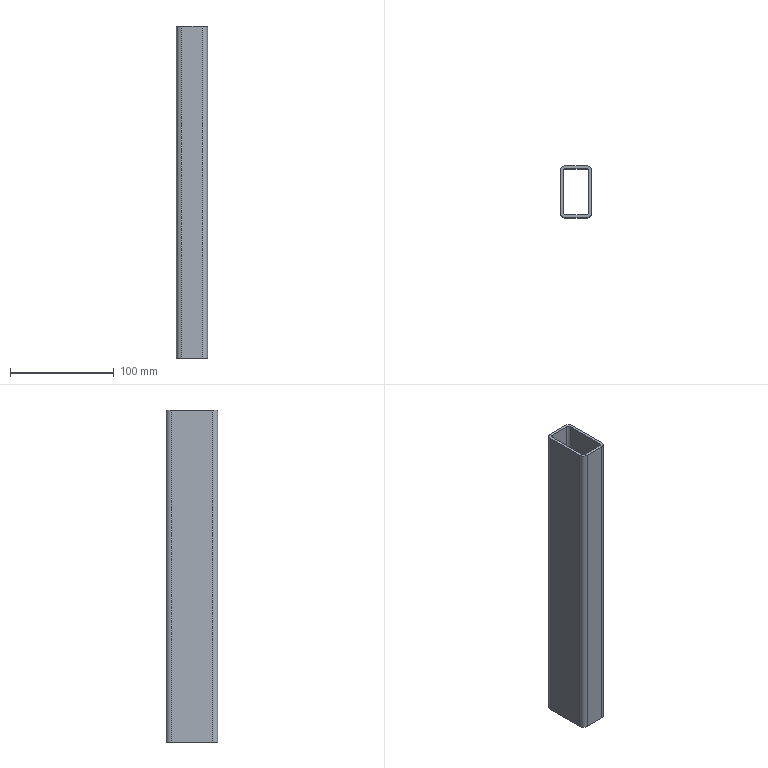Component | SolidWorks | Frame-1_SquareTube13-1 | 1 solid | 18 faces | box 30 x 50 x 320 mm | volume 118896 mm3 | plane 10 | cylinder 8 | commonest cylinder face diameters 5.2 x4 10.4 x4
STEP:
#1=COLOUR_RGB('',0.7922,0.8196,0.9333);
#2=FILL_AREA_STYLE_COLOUR('',#1);
#3=FILL_AREA_STYLE('',(#2));
#4=SURFACE_STYLE_FILL_AREA(#3);
#5=SURFACE_SIDE_STYLE('',(#4));
#6=SURFACE_STYLE_USAGE(.BOTH.,#5);
#7=PRESENTATION_STYLE_ASSIGNMENT((#6));
#8=CARTESIAN_POINT('',(-8.134,-11.622,-6.299));
#9=VERTEX_POINT('',#8);
#10=CARTESIAN_POINT('',(-8.134,-13.181,-6.299));
#11=VERTEX_POINT('',#10);
#12=CARTESIAN_POINT('',(-8.134,-11.622,-6.299));
#13=DIRECTION('',(0.,-1.,0.));
#14=VECTOR('',#13,39.37);
#15=LINE('',#12,#14);
#16=EDGE_CURVE('',#9,#11,#15,.T.);
#17=ORIENTED_EDGE('',*,*,#16,.T.);
#18=CARTESIAN_POINT('',(-8.134,-13.181,6.299));
#19=VERTEX_POINT('',#18);
#20=CARTESIAN_POINT('',(-8.134,-13.181,6.89));
#21=DIRECTION('',(0.,0.,1.));
#22=VECTOR('',#21,39.37);
#23=LINE('',#20,#22);
#24=EDGE_CURVE('',#11,#19,#23,.T.);
#25=ORIENTED_EDGE('',*,*,#24,.T.);
#26=CARTESIAN_POINT('',(-8.134,-11.622,6.299));
#27=VERTEX_POINT('',#26);
#28=CARTESIAN_POINT('',(-8.134,-11.622,6.299));
#29=DIRECTION('',(0.,1.,0.));
#30=VECTOR('',#29,39.37);
#31=LINE('',#28,#30);
#32=EDGE_CURVE('',#19,#27,#31,.T.);
#33=ORIENTED_EDGE('',*,*,#32,.T.);
#34=CARTESIAN_POINT('',(-8.134,-11.622,6.89));
#35=DIRECTION('',(-0.,0.,-1.));
#36=VECTOR('',#35,39.37);
#37=LINE('',#34,#36);
#38=EDGE_CURVE('',#27,#9,#37,.T.);
#39=ORIENTED_EDGE('',*,*,#38,.T.);
#40=EDGE_LOOP('',(#17,#25,#33,#39));
#41=FACE_OUTER_BOUND('',#40,.T.);
#42=CARTESIAN_POINT('',(-8.134,-11.622,6.89));
#43=DIRECTION('',(-1.,0.,0.));
#44=DIRECTION('',(0.,0.,1.));
#45=AXIS2_PLACEMENT_3D('',#42,#43,#44);
#46=PLANE('',#45);
#47=ADVANCED_FACE('',(#41),#46,.T.);
#48=ORIENTED_EDGE('',*,*,#24,.F.);
#49=CARTESIAN_POINT('',(-8.236,-13.283,-6.299));
#50=VERTEX_POINT('',#49);
#51=CARTESIAN_POINT('',(-8.236,-13.181,-6.299));
#52=DIRECTION('',(0.,0.,1.));
#53=DIRECTION('',(-1.,0.,0.));
#54=AXIS2_PLACEMENT_3D('',#51,#52,#53);
#55=CIRCLE('',#54,0.1024);
#56=EDGE_CURVE('',#50,#11,#55,.T.);
#57=ORIENTED_EDGE('',*,*,#56,.F.);
#58=CARTESIAN_POINT('',(-8.236,-13.283,6.299));
#59=VERTEX_POINT('',#58);
#60=CARTESIAN_POINT('',(-8.236,-13.283,6.89));
#61=DIRECTION('',(-0.,0.,-1.));
#62=VECTOR('',#61,39.37);
#63=LINE('',#60,#62);
#64=EDGE_CURVE('',#59,#50,#63,.T.);
#65=ORIENTED_EDGE('',*,*,#64,.F.);
#66=CARTESIAN_POINT('',(-8.236,-13.181,6.299));
#67=DIRECTION('',(-0.,0.,-1.));
#68=DIRECTION('',(-1.,0.,0.));
#69=AXIS2_PLACEMENT_3D('',#66,#67,#68);
#70=CIRCLE('',#69,0.1024);
#71=EDGE_CURVE('',#19,#59,#70,.T.);
#72=ORIENTED_EDGE('',*,*,#71,.F.);
#73=EDGE_LOOP('',(#48,#57,#65,#72));
#74=FACE_OUTER_BOUND('',#73,.T.);
#75=CARTESIAN_POINT('',(-8.236,-13.181,6.89));
#76=DIRECTION('',(-0.,0.,-1.));
#77=DIRECTION('',(-1.,0.,0.));
#78=AXIS2_PLACEMENT_3D('',#75,#76,#77);
#79=CYLINDRICAL_SURFACE('',#78,0.1024);
#80=ADVANCED_FACE('',(#74),#79,.F.);
#81=CARTESIAN_POINT('',(-8.236,-13.386,-6.299));
#82=VERTEX_POINT('',#81);
#83=CARTESIAN_POINT('',(-8.031,-13.181,-6.299));
#84=VERTEX_POINT('',#83);
#85=CARTESIAN_POINT('',(-8.236,-13.181,-6.299));
#86=DIRECTION('',(0.,0.,1.));
#87=DIRECTION('',(-1.,0.,0.));
#88=AXIS2_PLACEMENT_3D('',#85,#86,#87);
#89=CIRCLE('',#88,0.2047);
#90=EDGE_CURVE('',#82,#84,#89,.T.);
#91=ORIENTED_EDGE('',*,*,#90,.F.);
#92=CARTESIAN_POINT('',(-9.008,-13.386,-6.299));
#93=VERTEX_POINT('',#92);
#94=CARTESIAN_POINT('',(0.,-13.386,-6.299));
#95=DIRECTION('',(1.,0.,0.));
#96=VECTOR('',#95,39.37);
#97=LINE('',#94,#96);
#98=EDGE_CURVE('',#93,#82,#97,.T.);
#99=ORIENTED_EDGE('',*,*,#98,.F.);
#100=CARTESIAN_POINT('',(-9.213,-13.181,-6.299));
#101=VERTEX_POINT('',#100);
#102=CARTESIAN_POINT('',(-9.008,-13.181,-6.299));
#103=DIRECTION('',(0.,0.,1.));
#104=DIRECTION('',(-1.,0.,0.));
#105=AXIS2_PLACEMENT_3D('',#102,#103,#104);
#106=CIRCLE('',#105,0.2047);
#107=EDGE_CURVE('',#101,#93,#106,.T.);
#108=ORIENTED_EDGE('',*,*,#107,.F.);
#109=CARTESIAN_POINT('',(-9.213,-11.622,-6.299));
#110=VERTEX_POINT('',#109);
#111=CARTESIAN_POINT('',(-9.213,-12.402,-6.299));
#112=DIRECTION('',(0.,-1.,0.));
#113=VECTOR('',#112,39.37);
#114=LINE('',#111,#113);
#115=EDGE_CURVE('',#110,#101,#114,.T.);
#116=ORIENTED_EDGE('',*,*,#115,.F.);
#117=CARTESIAN_POINT('',(-9.008,-11.417,-6.299));
#118=VERTEX_POINT('',#117);
#119=CARTESIAN_POINT('',(-9.008,-11.622,-6.299));
#120=DIRECTION('',(0.,0.,1.));
#121=DIRECTION('',(-1.,0.,0.));
#122=AXIS2_PLACEMENT_3D('',#119,#120,#121);
#123=CIRCLE('',#122,0.2047);
#124=EDGE_CURVE('',#118,#110,#123,.T.);
#125=ORIENTED_EDGE('',*,*,#124,.F.);
#126=CARTESIAN_POINT('',(-8.236,-11.417,-6.299));
#127=VERTEX_POINT('',#126);
#128=CARTESIAN_POINT('',(0.,-11.417,-6.299));
#129=DIRECTION('',(-1.,0.,0.));
#130=VECTOR('',#129,39.37);
#131=LINE('',#128,#130);
#132=EDGE_CURVE('',#127,#118,#131,.T.);
#133=ORIENTED_EDGE('',*,*,#132,.F.);
#134=CARTESIAN_POINT('',(-8.031,-11.622,-6.299));
#135=VERTEX_POINT('',#134);
#136=CARTESIAN_POINT('',(-8.236,-11.622,-6.299));
#137=DIRECTION('',(0.,0.,1.));
#138=DIRECTION('',(-1.,0.,0.));
#139=AXIS2_PLACEMENT_3D('',#136,#137,#138);
#140=CIRCLE('',#139,0.2047);
#141=EDGE_CURVE('',#135,#127,#140,.T.);
#142=ORIENTED_EDGE('',*,*,#141,.F.);
#143=CARTESIAN_POINT('',(-8.031,-12.402,-6.299));
#144=DIRECTION('',(0.,1.,0.));
#145=VECTOR('',#144,39.37);
#146=LINE('',#143,#145);
#147=EDGE_CURVE('',#84,#135,#146,.T.);
#148=ORIENTED_EDGE('',*,*,#147,.F.);
#149=EDGE_LOOP('',(#91,#99,#108,#116,#125,#133,#142,#148));
#150=FACE_OUTER_BOUND('',#149,.T.);
#151=CARTESIAN_POINT('',(-9.11,-13.181,-6.299));
#152=VERTEX_POINT('',#151);
#153=CARTESIAN_POINT('',(-9.11,-11.622,-6.299));
#154=VERTEX_POINT('',#153);
#155=CARTESIAN_POINT('',(-9.11,-12.402,-6.299));
#156=DIRECTION('',(0.,1.,0.));
#157=VECTOR('',#156,39.37);
#158=LINE('',#155,#157);
#159=EDGE_CURVE('',#152,#154,#158,.T.);
#160=ORIENTED_EDGE('',*,*,#159,.F.);
#161=CARTESIAN_POINT('',(-9.008,-13.283,-6.299));
#162=VERTEX_POINT('',#161);
#163=CARTESIAN_POINT('',(-9.008,-13.181,-6.299));
#164=DIRECTION('',(-0.,0.,-1.));
#165=DIRECTION('',(-1.,0.,0.));
#166=AXIS2_PLACEMENT_3D('',#163,#164,#165);
#167=CIRCLE('',#166,0.1024);
#168=EDGE_CURVE('',#162,#152,#167,.T.);
#169=ORIENTED_EDGE('',*,*,#168,.F.);
#170=CARTESIAN_POINT('',(0.,-13.283,-6.299));
#171=DIRECTION('',(-1.,0.,0.));
#172=VECTOR('',#171,39.37);
#173=LINE('',#170,#172);
#174=EDGE_CURVE('',#50,#162,#173,.T.);
#175=ORIENTED_EDGE('',*,*,#174,.F.);
#176=ORIENTED_EDGE('',*,*,#56,.T.);
#177=ORIENTED_EDGE('',*,*,#16,.F.);
#178=CARTESIAN_POINT('',(-8.236,-11.52,-6.299));
#179=VERTEX_POINT('',#178);
#180=CARTESIAN_POINT('',(-8.236,-11.622,-6.299));
#181=DIRECTION('',(-0.,0.,-1.));
#182=DIRECTION('',(-1.,0.,0.));
#183=AXIS2_PLACEMENT_3D('',#180,#181,#182);
#184=CIRCLE('',#183,0.1024);
#185=EDGE_CURVE('',#179,#9,#184,.T.);
#186=ORIENTED_EDGE('',*,*,#185,.F.);
#187=CARTESIAN_POINT('',(-9.008,-11.52,-6.299));
#188=VERTEX_POINT('',#187);
#189=CARTESIAN_POINT('',(0.,-11.52,-6.299));
#190=DIRECTION('',(1.,0.,0.));
#191=VECTOR('',#190,39.37);
#192=LINE('',#189,#191);
#193=EDGE_CURVE('',#188,#179,#192,.T.);
#194=ORIENTED_EDGE('',*,*,#193,.F.);
#195=CARTESIAN_POINT('',(-9.008,-11.622,-6.299));
#196=DIRECTION('',(-0.,0.,-1.));
#197=DIRECTION('',(-1.,0.,0.));
#198=AXIS2_PLACEMENT_3D('',#195,#196,#197);
#199=CIRCLE('',#198,0.1024);
#200=EDGE_CURVE('',#154,#188,#199,.T.);
#201=ORIENTED_EDGE('',*,*,#200,.F.);
#202=EDGE_LOOP('',(#160,#169,#175,#176,#177,#186,#194,#201));
#203=FACE_BOUND('',#202,.T.);
#204=CARTESIAN_POINT('',(0.,-12.402,-6.299));
#205=DIRECTION('',(0.,0.,1.));
#206=DIRECTION('',(1.,0.,0.));
#207=AXIS2_PLACEMENT_3D('',#204,#205,#206);
#208=PLANE('',#207);
#209=ADVANCED_FACE('',(#150,#203),#208,.F.);
#210=CARTESIAN_POINT('',(-8.236,-11.52,6.299));
#211=VERTEX_POINT('',#210);
#212=CARTESIAN_POINT('',(-8.236,-11.52,6.89));
#213=DIRECTION('',(0.,0.,1.));
#214=VECTOR('',#213,39.37);
#215=LINE('',#212,#214);
#216=EDGE_CURVE('',#179,#211,#215,.T.);
#217=ORIENTED_EDGE('',*,*,#216,.F.);
#218=ORIENTED_EDGE('',*,*,#185,.T.);
#219=ORIENTED_EDGE('',*,*,#38,.F.);
#220=CARTESIAN_POINT('',(-8.236,-11.622,6.299));
#221=DIRECTION('',(-0.,0.,-1.));
#222=DIRECTION('',(-1.,0.,0.));
#223=AXIS2_PLACEMENT_3D('',#220,#221,#222);
#224=CIRCLE('',#223,0.1024);
#225=EDGE_CURVE('',#211,#27,#224,.T.);
#226=ORIENTED_EDGE('',*,*,#225,.F.);
#227=EDGE_LOOP('',(#217,#218,#219,#226));
#228=FACE_OUTER_BOUND('',#227,.T.);
#229=CARTESIAN_POINT('',(-8.236,-11.622,6.89));
#230=DIRECTION('',(-0.,0.,-1.));
#231=DIRECTION('',(-1.,0.,0.));
#232=AXIS2_PLACEMENT_3D('',#229,#230,#231);
#233=CYLINDRICAL_SURFACE('',#232,0.1024);
#234=ADVANCED_FACE('',(#228),#233,.F.);
#235=CARTESIAN_POINT('',(-9.008,-11.417,6.299));
#236=VERTEX_POINT('',#235);
#237=CARTESIAN_POINT('',(-8.236,-11.417,6.299));
#238=VERTEX_POINT('',#237);
#239=CARTESIAN_POINT('',(0.,-11.417,6.299));
#240=DIRECTION('',(1.,0.,0.));
#241=VECTOR('',#240,39.37);
#242=LINE('',#239,#241);
#243=EDGE_CURVE('',#236,#238,#242,.T.);
#244=ORIENTED_EDGE('',*,*,#243,.F.);
#245=CARTESIAN_POINT('',(-9.213,-11.622,6.299));
#246=VERTEX_POINT('',#245);
#247=CARTESIAN_POINT('',(-9.008,-11.622,6.299));
#248=DIRECTION('',(-0.,0.,-1.));
#249=DIRECTION('',(-1.,0.,0.));
#250=AXIS2_PLACEMENT_3D('',#247,#248,#249);
#251=CIRCLE('',#250,0.2047);
#252=EDGE_CURVE('',#246,#236,#251,.T.);
#253=ORIENTED_EDGE('',*,*,#252,.F.);
#254=CARTESIAN_POINT('',(-9.213,-13.181,6.299));
#255=VERTEX_POINT('',#254);
#256=CARTESIAN_POINT('',(-9.213,-12.402,6.299));
#257=DIRECTION('',(0.,1.,0.));
#258=VECTOR('',#257,39.37);
#259=LINE('',#256,#258);
#260=EDGE_CURVE('',#255,#246,#259,.T.);
#261=ORIENTED_EDGE('',*,*,#260,.F.);
#262=CARTESIAN_POINT('',(-9.008,-13.386,6.299));
#263=VERTEX_POINT('',#262);
#264=CARTESIAN_POINT('',(-9.008,-13.181,6.299));
#265=DIRECTION('',(-0.,0.,-1.));
#266=DIRECTION('',(-1.,0.,0.));
#267=AXIS2_PLACEMENT_3D('',#264,#265,#266);
#268=CIRCLE('',#267,0.2047);
#269=EDGE_CURVE('',#263,#255,#268,.T.);
#270=ORIENTED_EDGE('',*,*,#269,.F.);
#271=CARTESIAN_POINT('',(-8.236,-13.386,6.299));
#272=VERTEX_POINT('',#271);
#273=CARTESIAN_POINT('',(0.,-13.386,6.299));
#274=DIRECTION('',(-1.,0.,0.));
#275=VECTOR('',#274,39.37);
#276=LINE('',#273,#275);
#277=EDGE_CURVE('',#272,#263,#276,.T.);
#278=ORIENTED_EDGE('',*,*,#277,.F.);
#279=CARTESIAN_POINT('',(-8.031,-13.181,6.299));
#280=VERTEX_POINT('',#279);
#281=CARTESIAN_POINT('',(-8.236,-13.181,6.299));
#282=DIRECTION('',(-0.,0.,-1.));
#283=DIRECTION('',(-1.,0.,0.));
#284=AXIS2_PLACEMENT_3D('',#281,#282,#283);
#285=CIRCLE('',#284,0.2047);
#286=EDGE_CURVE('',#280,#272,#285,.T.);
#287=ORIENTED_EDGE('',*,*,#286,.F.);
#288=CARTESIAN_POINT('',(-8.031,-11.622,6.299));
#289=VERTEX_POINT('',#288);
#290=CARTESIAN_POINT('',(-8.031,-12.402,6.299));
#291=DIRECTION('',(0.,-1.,0.));
#292=VECTOR('',#291,39.37);
#293=LINE('',#290,#292);
#294=EDGE_CURVE('',#289,#280,#293,.T.);
#295=ORIENTED_EDGE('',*,*,#294,.F.);
#296=CARTESIAN_POINT('',(-8.236,-11.622,6.299));
#297=DIRECTION('',(-0.,0.,-1.));
#298=DIRECTION('',(-1.,0.,0.));
#299=AXIS2_PLACEMENT_3D('',#296,#297,#298);
#300=CIRCLE('',#299,0.2047);
#301=EDGE_CURVE('',#238,#289,#300,.T.);
#302=ORIENTED_EDGE('',*,*,#301,.F.);
#303=EDGE_LOOP('',(#244,#253,#261,#270,#278,#287,#295,#302));
#304=FACE_OUTER_BOUND('',#303,.T.);
#305=CARTESIAN_POINT('',(-9.008,-11.52,6.299));
#306=VERTEX_POINT('',#305);
#307=CARTESIAN_POINT('',(-9.11,-11.622,6.299));
#308=VERTEX_POINT('',#307);
#309=CARTESIAN_POINT('',(-9.008,-11.622,6.299));
#310=DIRECTION('',(0.,0.,1.));
#311=DIRECTION('',(-1.,0.,0.));
#312=AXIS2_PLACEMENT_3D('',#309,#310,#311);
#313=CIRCLE('',#312,0.1024);
#314=EDGE_CURVE('',#306,#308,#313,.T.);
#315=ORIENTED_EDGE('',*,*,#314,.F.);
#316=CARTESIAN_POINT('',(0.,-11.52,6.299));
#317=DIRECTION('',(-1.,0.,0.));
#318=VECTOR('',#317,39.37);
#319=LINE('',#316,#318);
#320=EDGE_CURVE('',#211,#306,#319,.T.);
#321=ORIENTED_EDGE('',*,*,#320,.F.);
#322=ORIENTED_EDGE('',*,*,#225,.T.);
#323=ORIENTED_EDGE('',*,*,#32,.F.);
#324=ORIENTED_EDGE('',*,*,#71,.T.);
#325=CARTESIAN_POINT('',(-9.008,-13.283,6.299));
#326=VERTEX_POINT('',#325);
#327=CARTESIAN_POINT('',(0.,-13.283,6.299));
#328=DIRECTION('',(1.,0.,0.));
#329=VECTOR('',#328,39.37);
#330=LINE('',#327,#329);
#331=EDGE_CURVE('',#326,#59,#330,.T.);
#332=ORIENTED_EDGE('',*,*,#331,.F.);
#333=CARTESIAN_POINT('',(-9.11,-13.181,6.299));
#334=VERTEX_POINT('',#333);
#335=CARTESIAN_POINT('',(-9.008,-13.181,6.299));
#336=DIRECTION('',(0.,0.,1.));
#337=DIRECTION('',(-1.,0.,0.));
#338=AXIS2_PLACEMENT_3D('',#335,#336,#337);
#339=CIRCLE('',#338,0.1024);
#340=EDGE_CURVE('',#334,#326,#339,.T.);
#341=ORIENTED_EDGE('',*,*,#340,.F.);
#342=CARTESIAN_POINT('',(-9.11,-12.402,6.299));
#343=DIRECTION('',(0.,-1.,0.));
#344=VECTOR('',#343,39.37);
#345=LINE('',#342,#344);
#346=EDGE_CURVE('',#308,#334,#345,.T.);
#347=ORIENTED_EDGE('',*,*,#346,.F.);
#348=EDGE_LOOP('',(#315,#321,#322,#323,#324,#332,#341,#347));
#349=FACE_BOUND('',#348,.T.);
#350=CARTESIAN_POINT('',(0.,-12.402,6.299));
#351=DIRECTION('',(0.,0.,-1.));
#352=DIRECTION('',(-1.,0.,0.));
#353=AXIS2_PLACEMENT_3D('',#350,#351,#352);
#354=PLANE('',#353);
#355=ADVANCED_FACE('',(#304,#349),#354,.F.);
#356=ORIENTED_EDGE('',*,*,#174,.T.);
#357=CARTESIAN_POINT('',(-9.008,-13.283,6.89));
#358=DIRECTION('',(0.,0.,1.));
#359=VECTOR('',#358,39.37);
#360=LINE('',#357,#359);
#361=EDGE_CURVE('',#162,#326,#360,.T.);
#362=ORIENTED_EDGE('',*,*,#361,.T.);
#363=ORIENTED_EDGE('',*,*,#331,.T.);
#364=ORIENTED_EDGE('',*,*,#64,.T.);
#365=EDGE_LOOP('',(#356,#362,#363,#364));
#366=FACE_OUTER_BOUND('',#365,.T.);
#367=CARTESIAN_POINT('',(-9.008,-13.283,6.89));
#368=DIRECTION('',(0.,1.,0.));
#369=DIRECTION('',(0.,0.,1.));
#370=AXIS2_PLACEMENT_3D('',#367,#368,#369);
#371=PLANE('',#370);
#372=ADVANCED_FACE('',(#366),#371,.T.);
#373=ORIENTED_EDGE('',*,*,#294,.T.);
#374=CARTESIAN_POINT('',(-8.031,-13.181,6.89));
#375=DIRECTION('',(0.,0.,1.));
#376=VECTOR('',#375,39.37);
#377=LINE('',#374,#376);
#378=EDGE_CURVE('',#84,#280,#377,.T.);
#379=ORIENTED_EDGE('',*,*,#378,.F.);
#380=ORIENTED_EDGE('',*,*,#147,.T.);
#381=CARTESIAN_POINT('',(-8.031,-11.622,6.89));
#382=DIRECTION('',(-0.,0.,-1.));
#383=VECTOR('',#382,39.37);
#384=LINE('',#381,#383);
#385=EDGE_CURVE('',#289,#135,#384,.T.);
#386=ORIENTED_EDGE('',*,*,#385,.F.);
#387=EDGE_LOOP('',(#373,#379,#380,#386));
#388=FACE_OUTER_BOUND('',#387,.T.);
#389=CARTESIAN_POINT('',(-8.031,-11.622,6.89));
#390=DIRECTION('',(-1.,0.,0.));
#391=DIRECTION('',(0.,0.,1.));
#392=AXIS2_PLACEMENT_3D('',#389,#390,#391);
#393=PLANE('',#392);
#394=ADVANCED_FACE('',(#388),#393,.F.);
#395=CARTESIAN_POINT('',(-8.236,-13.386,6.89));
#396=DIRECTION('',(-0.,0.,-1.));
#397=VECTOR('',#396,39.37);
#398=LINE('',#395,#397);
#399=EDGE_CURVE('',#272,#82,#398,.T.);
#400=ORIENTED_EDGE('',*,*,#399,.T.);
#401=ORIENTED_EDGE('',*,*,#90,.T.);
#402=ORIENTED_EDGE('',*,*,#378,.T.);
#403=ORIENTED_EDGE('',*,*,#286,.T.);
#404=EDGE_LOOP('',(#400,#401,#402,#403));
#405=FACE_OUTER_BOUND('',#404,.T.);
#406=CARTESIAN_POINT('',(-8.236,-13.181,6.89));
#407=DIRECTION('',(-0.,0.,-1.));
#408=DIRECTION('',(-1.,0.,0.));
#409=AXIS2_PLACEMENT_3D('',#406,#407,#408);
#410=CYLINDRICAL_SURFACE('',#409,0.2047);
#411=ADVANCED_FACE('',(#405),#410,.T.);
#412=ORIENTED_EDGE('',*,*,#277,.T.);
#413=CARTESIAN_POINT('',(-9.008,-13.386,6.89));
#414=DIRECTION('',(0.,0.,1.));
#415=VECTOR('',#414,39.37);
#416=LINE('',#413,#415);
#417=EDGE_CURVE('',#93,#263,#416,.T.);
#418=ORIENTED_EDGE('',*,*,#417,.F.);
#419=ORIENTED_EDGE('',*,*,#98,.T.);
#420=ORIENTED_EDGE('',*,*,#399,.F.);
#421=EDGE_LOOP('',(#412,#418,#419,#420));
#422=FACE_OUTER_BOUND('',#421,.T.);
#423=CARTESIAN_POINT('',(-9.008,-13.386,6.89));
#424=DIRECTION('',(0.,1.,0.));
#425=DIRECTION('',(0.,0.,1.));
#426=AXIS2_PLACEMENT_3D('',#423,#424,#425);
#427=PLANE('',#426);
#428=ADVANCED_FACE('',(#422),#427,.F.);
#429=CARTESIAN_POINT('',(-9.213,-13.181,6.89));
#430=DIRECTION('',(-0.,0.,-1.));
#431=VECTOR('',#430,39.37);
#432=LINE('',#429,#431);
#433=EDGE_CURVE('',#255,#101,#432,.T.);
#434=ORIENTED_EDGE('',*,*,#433,.T.);
#435=ORIENTED_EDGE('',*,*,#107,.T.);
#436=ORIENTED_EDGE('',*,*,#417,.T.);
#437=ORIENTED_EDGE('',*,*,#269,.T.);
#438=EDGE_LOOP('',(#434,#435,#436,#437));
#439=FACE_OUTER_BOUND('',#438,.T.);
#440=CARTESIAN_POINT('',(-9.008,-13.181,6.89));
#441=DIRECTION('',(-0.,0.,-1.));
#442=DIRECTION('',(-1.,0.,0.));
#443=AXIS2_PLACEMENT_3D('',#440,#441,#442);
#444=CYLINDRICAL_SURFACE('',#443,0.2047);
#445=ADVANCED_FACE('',(#439),#444,.T.);
#446=ORIENTED_EDGE('',*,*,#260,.T.);
#447=CARTESIAN_POINT('',(-9.213,-11.622,6.89));
#448=DIRECTION('',(0.,0.,1.));
#449=VECTOR('',#448,39.37);
#450=LINE('',#447,#449);
#451=EDGE_CURVE('',#110,#246,#450,.T.);
#452=ORIENTED_EDGE('',*,*,#451,.F.);
#453=ORIENTED_EDGE('',*,*,#115,.T.);
#454=ORIENTED_EDGE('',*,*,#433,.F.);
#455=EDGE_LOOP('',(#446,#452,#453,#454));
#456=FACE_OUTER_BOUND('',#455,.T.);
#457=CARTESIAN_POINT('',(-9.213,-13.181,6.89));
#458=DIRECTION('',(1.,0.,-0.));
#459=DIRECTION('',(-0.,0.,-1.));
#460=AXIS2_PLACEMENT_3D('',#457,#458,#459);
#461=PLANE('',#460);
#462=ADVANCED_FACE('',(#456),#461,.F.);
#463=CARTESIAN_POINT('',(-9.008,-11.417,6.89));
#464=DIRECTION('',(-0.,0.,-1.));
#465=VECTOR('',#464,39.37);
#466=LINE('',#463,#465);
#467=EDGE_CURVE('',#236,#118,#466,.T.);
#468=ORIENTED_EDGE('',*,*,#467,.T.);
#469=ORIENTED_EDGE('',*,*,#124,.T.);
#470=ORIENTED_EDGE('',*,*,#451,.T.);
#471=ORIENTED_EDGE('',*,*,#252,.T.);
#472=EDGE_LOOP('',(#468,#469,#470,#471));
#473=FACE_OUTER_BOUND('',#472,.T.);
#474=CARTESIAN_POINT('',(-9.008,-11.622,6.89));
#475=DIRECTION('',(-0.,0.,-1.));
#476=DIRECTION('',(-1.,0.,0.));
#477=AXIS2_PLACEMENT_3D('',#474,#475,#476);
#478=CYLINDRICAL_SURFACE('',#477,0.2047);
#479=ADVANCED_FACE('',(#473),#478,.T.);
#480=ORIENTED_EDGE('',*,*,#243,.T.);
#481=CARTESIAN_POINT('',(-8.236,-11.417,6.89));
#482=DIRECTION('',(0.,0.,1.));
#483=VECTOR('',#482,39.37);
#484=LINE('',#481,#483);
#485=EDGE_CURVE('',#127,#238,#484,.T.);
#486=ORIENTED_EDGE('',*,*,#485,.F.);
#487=ORIENTED_EDGE('',*,*,#132,.T.);
#488=ORIENTED_EDGE('',*,*,#467,.F.);
#489=EDGE_LOOP('',(#480,#486,#487,#488));
#490=FACE_OUTER_BOUND('',#489,.T.);
#491=CARTESIAN_POINT('',(-8.236,-11.417,6.89));
#492=DIRECTION('',(0.,-1.,0.));
#493=DIRECTION('',(0.,0.,-1.));
#494=AXIS2_PLACEMENT_3D('',#491,#492,#493);
#495=PLANE('',#494);
#496=ADVANCED_FACE('',(#490),#495,.F.);
#497=ORIENTED_EDGE('',*,*,#385,.T.);
#498=ORIENTED_EDGE('',*,*,#141,.T.);
#499=ORIENTED_EDGE('',*,*,#485,.T.);
#500=ORIENTED_EDGE('',*,*,#301,.T.);
#501=EDGE_LOOP('',(#497,#498,#499,#500));
#502=FACE_OUTER_BOUND('',#501,.T.);
#503=CARTESIAN_POINT('',(-8.236,-11.622,6.89));
#504=DIRECTION('',(-0.,0.,-1.));
#505=DIRECTION('',(-1.,0.,0.));
#506=AXIS2_PLACEMENT_3D('',#503,#504,#505);
#507=CYLINDRICAL_SURFACE('',#506,0.2047);
#508=ADVANCED_FACE('',(#502),#507,.T.);
#509=CARTESIAN_POINT('',(-9.11,-11.622,6.89));
#510=DIRECTION('',(0.,0.,1.));
#511=VECTOR('',#510,39.37);
#512=LINE('',#509,#511);
#513=EDGE_CURVE('',#154,#308,#512,.T.);
#514=ORIENTED_EDGE('',*,*,#513,.F.);
#515=ORIENTED_EDGE('',*,*,#200,.T.);
#516=CARTESIAN_POINT('',(-9.008,-11.52,6.89));
#517=DIRECTION('',(-0.,0.,-1.));
#518=VECTOR('',#517,39.37);
#519=LINE('',#516,#518);
#520=EDGE_CURVE('',#306,#188,#519,.T.);
#521=ORIENTED_EDGE('',*,*,#520,.F.);
#522=ORIENTED_EDGE('',*,*,#314,.T.);
#523=EDGE_LOOP('',(#514,#515,#521,#522));
#524=FACE_OUTER_BOUND('',#523,.T.);
#525=CARTESIAN_POINT('',(-9.008,-11.622,6.89));
#526=DIRECTION('',(-0.,0.,-1.));
#527=DIRECTION('',(-1.,0.,0.));
#528=AXIS2_PLACEMENT_3D('',#525,#526,#527);
#529=CYLINDRICAL_SURFACE('',#528,0.1024);
#530=ADVANCED_FACE('',(#524),#529,.F.);
#531=ORIENTED_EDGE('',*,*,#159,.T.);
#532=ORIENTED_EDGE('',*,*,#513,.T.);
#533=ORIENTED_EDGE('',*,*,#346,.T.);
#534=CARTESIAN_POINT('',(-9.11,-13.181,6.89));
#535=DIRECTION('',(-0.,0.,-1.));
#536=VECTOR('',#535,39.37);
#537=LINE('',#534,#536);
#538=EDGE_CURVE('',#334,#152,#537,.T.);
#539=ORIENTED_EDGE('',*,*,#538,.T.);
#540=EDGE_LOOP('',(#531,#532,#533,#539));
#541=FACE_OUTER_BOUND('',#540,.T.);
#542=CARTESIAN_POINT('',(-9.11,-13.181,6.89));
#543=DIRECTION('',(1.,0.,-0.));
#544=DIRECTION('',(-0.,0.,-1.));
#545=AXIS2_PLACEMENT_3D('',#542,#543,#544);
#546=PLANE('',#545);
#547=ADVANCED_FACE('',(#541),#546,.T.);
#548=ORIENTED_EDGE('',*,*,#361,.F.);
#549=ORIENTED_EDGE('',*,*,#168,.T.);
#550=ORIENTED_EDGE('',*,*,#538,.F.);
#551=ORIENTED_EDGE('',*,*,#340,.T.);
#552=EDGE_LOOP('',(#548,#549,#550,#551));
#553=FACE_OUTER_BOUND('',#552,.T.);
#554=CARTESIAN_POINT('',(-9.008,-13.181,6.89));
#555=DIRECTION('',(-0.,0.,-1.));
#556=DIRECTION('',(-1.,0.,0.));
#557=AXIS2_PLACEMENT_3D('',#554,#555,#556);
#558=CYLINDRICAL_SURFACE('',#557,0.1024);
#559=ADVANCED_FACE('',(#553),#558,.F.);
#560=ORIENTED_EDGE('',*,*,#193,.T.);
#561=ORIENTED_EDGE('',*,*,#216,.T.);
#562=ORIENTED_EDGE('',*,*,#320,.T.);
#563=ORIENTED_EDGE('',*,*,#520,.T.);
#564=EDGE_LOOP('',(#560,#561,#562,#563));
#565=FACE_OUTER_BOUND('',#564,.T.);
#566=CARTESIAN_POINT('',(-8.236,-11.52,6.89));
#567=DIRECTION('',(0.,-1.,0.));
#568=DIRECTION('',(0.,0.,-1.));
#569=AXIS2_PLACEMENT_3D('',#566,#567,#568);
#570=PLANE('',#569);
#571=ADVANCED_FACE('',(#565),#570,.T.);
#572=CLOSED_SHELL('',(#47,#80,#209,#234,#355,#372,#394,#411,#428,#445,#462,#479,#496,#508,#530,#547,#559,#571));
#573=MANIFOLD_SOLID_BREP('',#572);
#574=STYLED_ITEM('',(#7),#573);
#575=(LENGTH_UNIT()NAMED_UNIT(*)SI_UNIT($,.METRE.));
#576=LENGTH_MEASURE_WITH_UNIT(LENGTH_MEASURE(0.0254),#575);
#577=DIMENSIONAL_EXPONENTS(1.,0.,0.,0.,0.,0.,0.);
#578=(CONVERSION_BASED_UNIT('',#576)LENGTH_UNIT()NAMED_UNIT(#577));
#579=UNCERTAINTY_MEASURE_WITH_UNIT(LENGTH_MEASURE(0.00001),#578,'','');
#580=(NAMED_UNIT(*)PLANE_ANGLE_UNIT()SI_UNIT($,.RADIAN.));
#581=(NAMED_UNIT(*)SI_UNIT($,.STERADIAN.)SOLID_ANGLE_UNIT());
#582=(GEOMETRIC_REPRESENTATION_CONTEXT(3)GLOBAL_UNCERTAINTY_ASSIGNED_CONTEXT((#579))GLOBAL_UNIT_ASSIGNED_CONTEXT((#578,#580,#581))REPRESENTATION_CONTEXT('',''));
#583=MECHANICAL_DESIGN_GEOMETRIC_PRESENTATION_REPRESENTATION('',(#574),#582);
#584=PRESENTATION_LAYER_ASSIGNMENT('','',(#574));
#585=CARTESIAN_POINT('',(0.,0.,0.));
#586=DIRECTION('',(0.,0.,1.));
#587=DIRECTION('',(1.,0.,0.));
#588=AXIS2_PLACEMENT_3D('',#585,#586,#587);
#589=(LENGTH_UNIT()NAMED_UNIT(*)SI_UNIT($,.METRE.));
#590=LENGTH_MEASURE_WITH_UNIT(LENGTH_MEASURE(0.0254),#589);
#591=DIMENSIONAL_EXPONENTS(1.,0.,0.,0.,0.,0.,0.);
#592=(CONVERSION_BASED_UNIT('',#590)LENGTH_UNIT()NAMED_UNIT(#591));
#593=UNCERTAINTY_MEASURE_WITH_UNIT(LENGTH_MEASURE(0.00001),#592,'','');
#594=(NAMED_UNIT(*)PLANE_ANGLE_UNIT()SI_UNIT($,.RADIAN.));
#595=(NAMED_UNIT(*)SI_UNIT($,.STERADIAN.)SOLID_ANGLE_UNIT());
#596=(GEOMETRIC_REPRESENTATION_CONTEXT(3)GLOBAL_UNCERTAINTY_ASSIGNED_CONTEXT((#593))GLOBAL_UNIT_ASSIGNED_CONTEXT((#592,#594,#595))REPRESENTATION_CONTEXT('',''));
#597=ADVANCED_BREP_SHAPE_REPRESENTATION('',(#573,#588),#596);